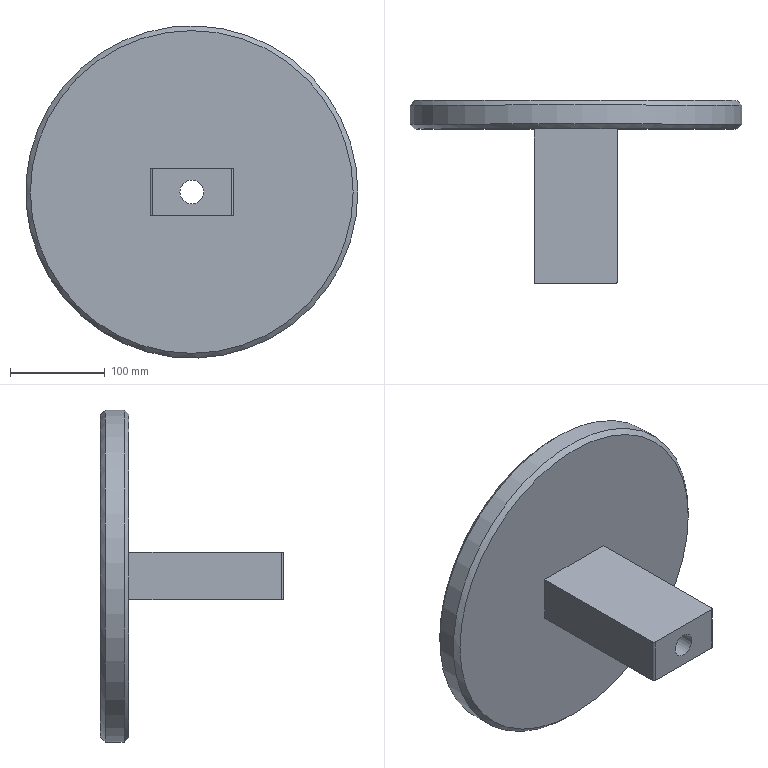Component | NX | PUNCH | 1 solid | 25 faces | volume 3459497 mm3 | cone 10 | cylinder 8 | plane 7 | commonest cylinder face diameters 14 x4 4 x2 350 x1 25 x1